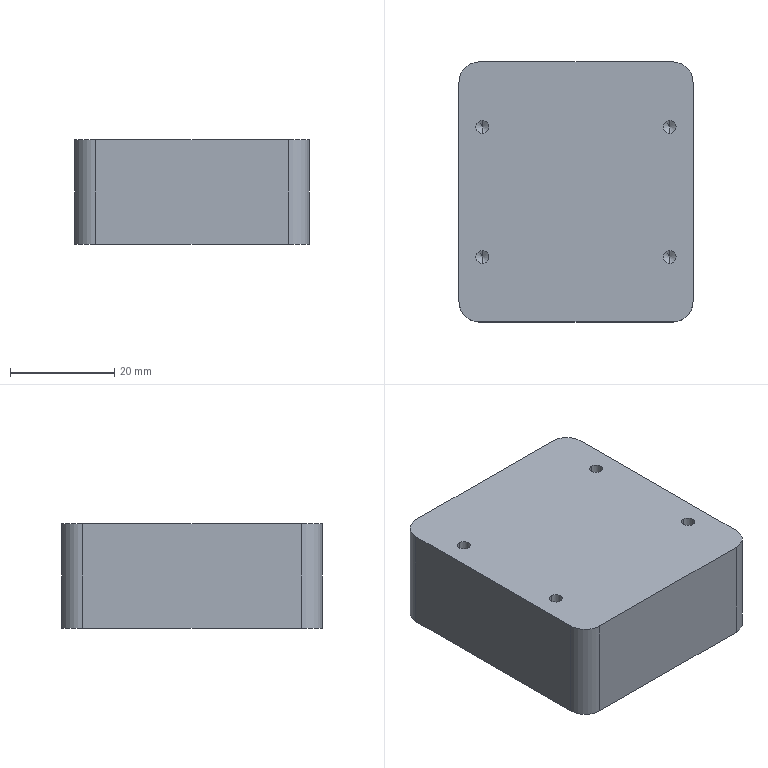CAM job | Mastercam | mm | 8 operations | part box 45 x 50 x 20
1. Facing | 24 - 100 平铣刀
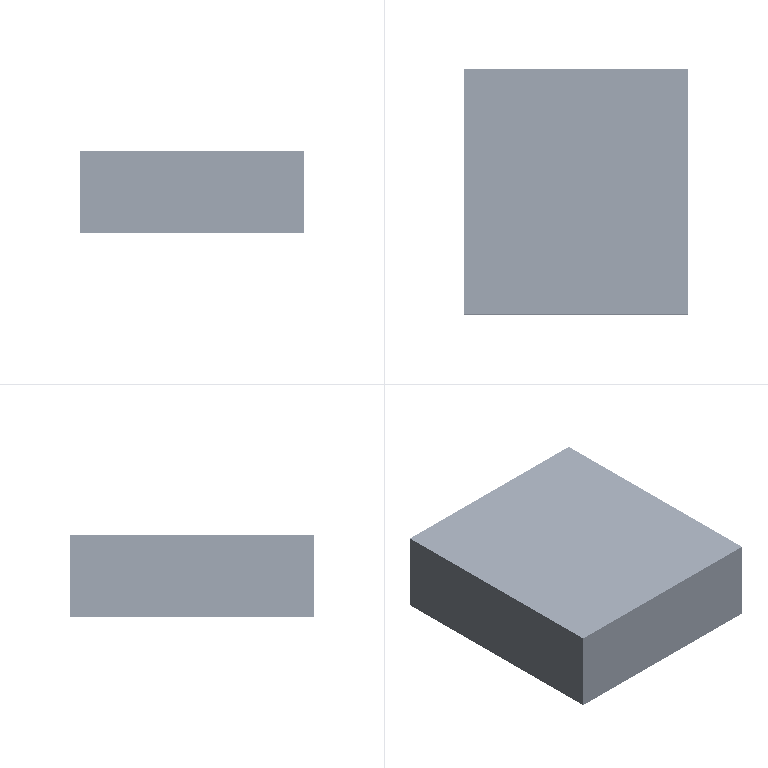2. Contour (Ramp) | 10 - 10 平铣刀
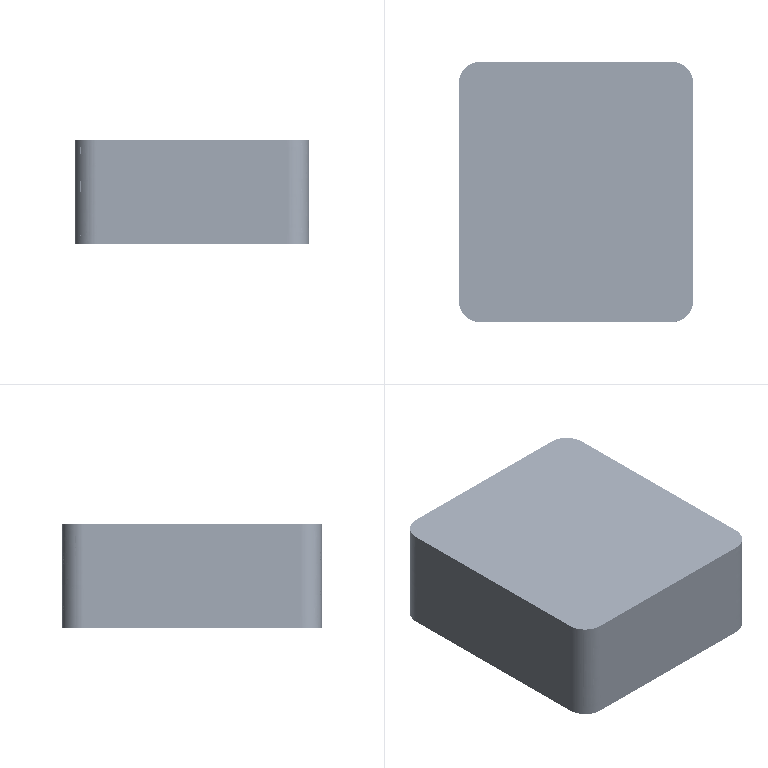3. Contour (2D) | 10 - 10 平铣刀
4. Contour (2D chamfer) | 7 - 4 倒角刀
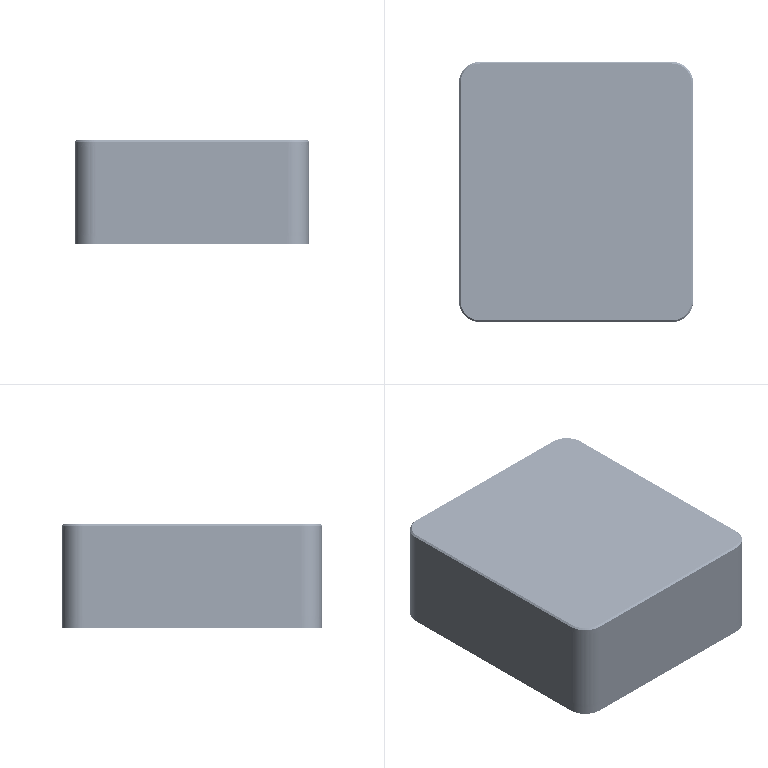5. Drill/Counterbore | 7 - 4 倒角刀
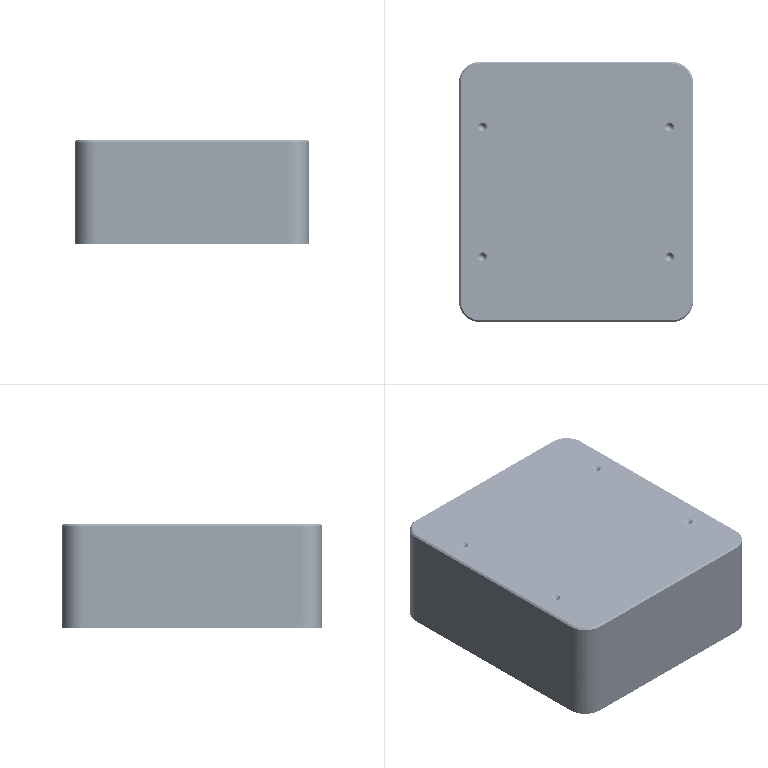6. Facing | 24 - 100 平铣刀
7. Contour (2D chamfer) | 7 - 4 倒角刀
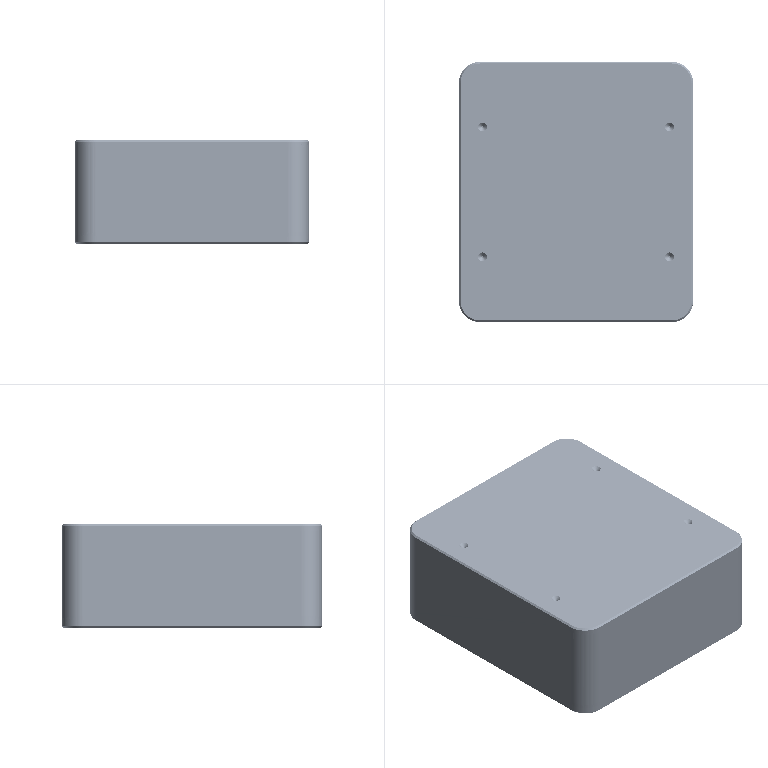8. Drill/Counterbore | 7 - 4 倒角刀